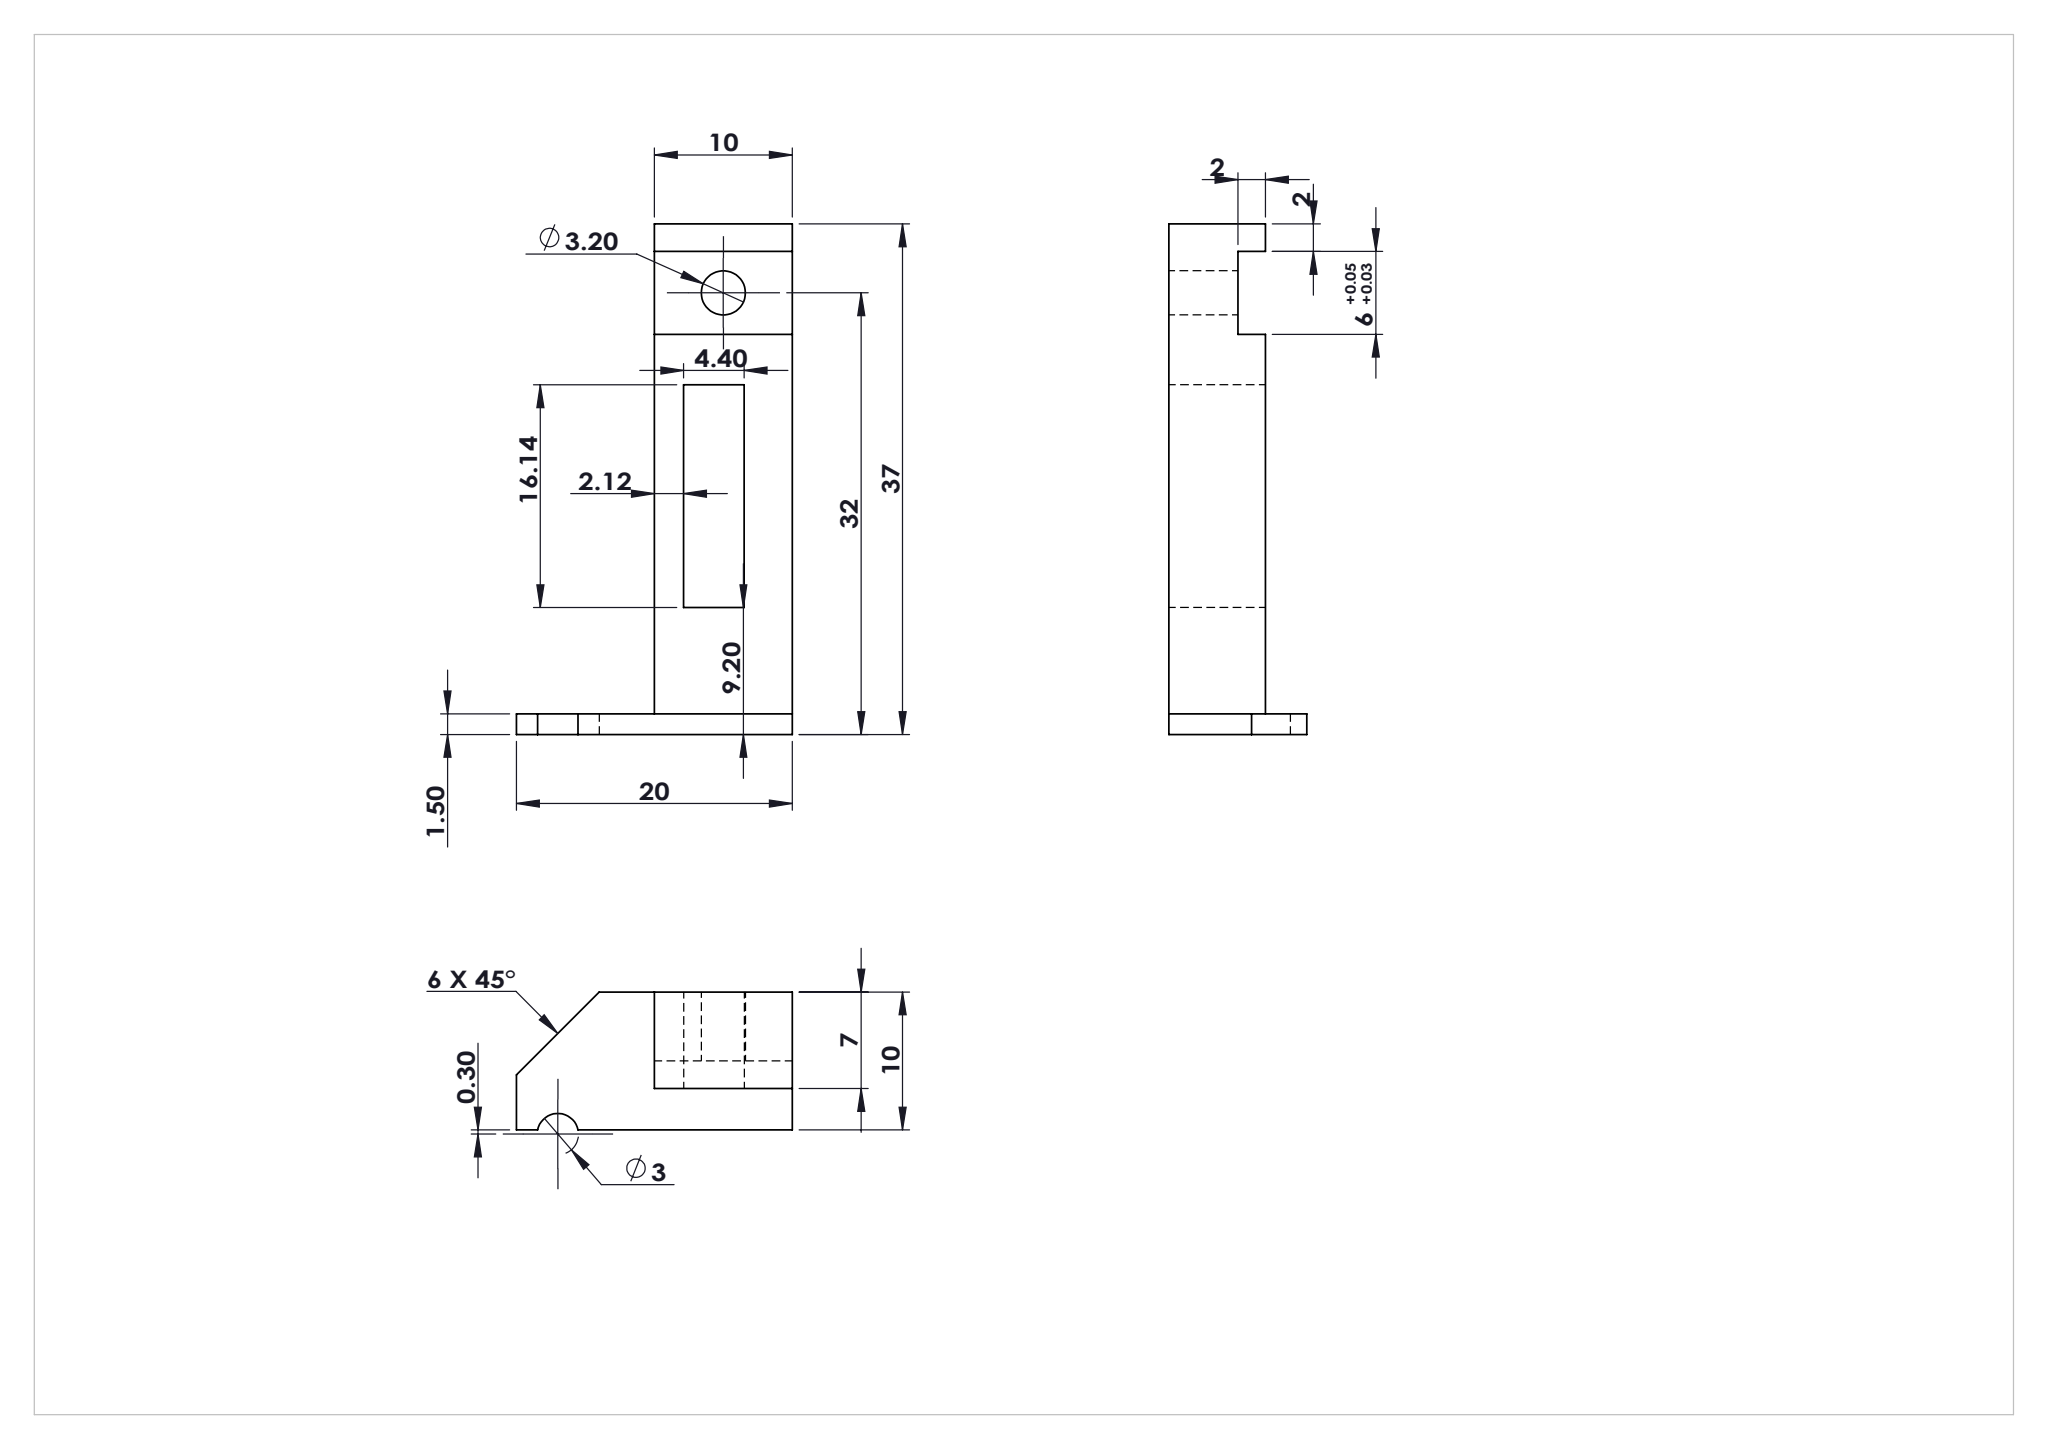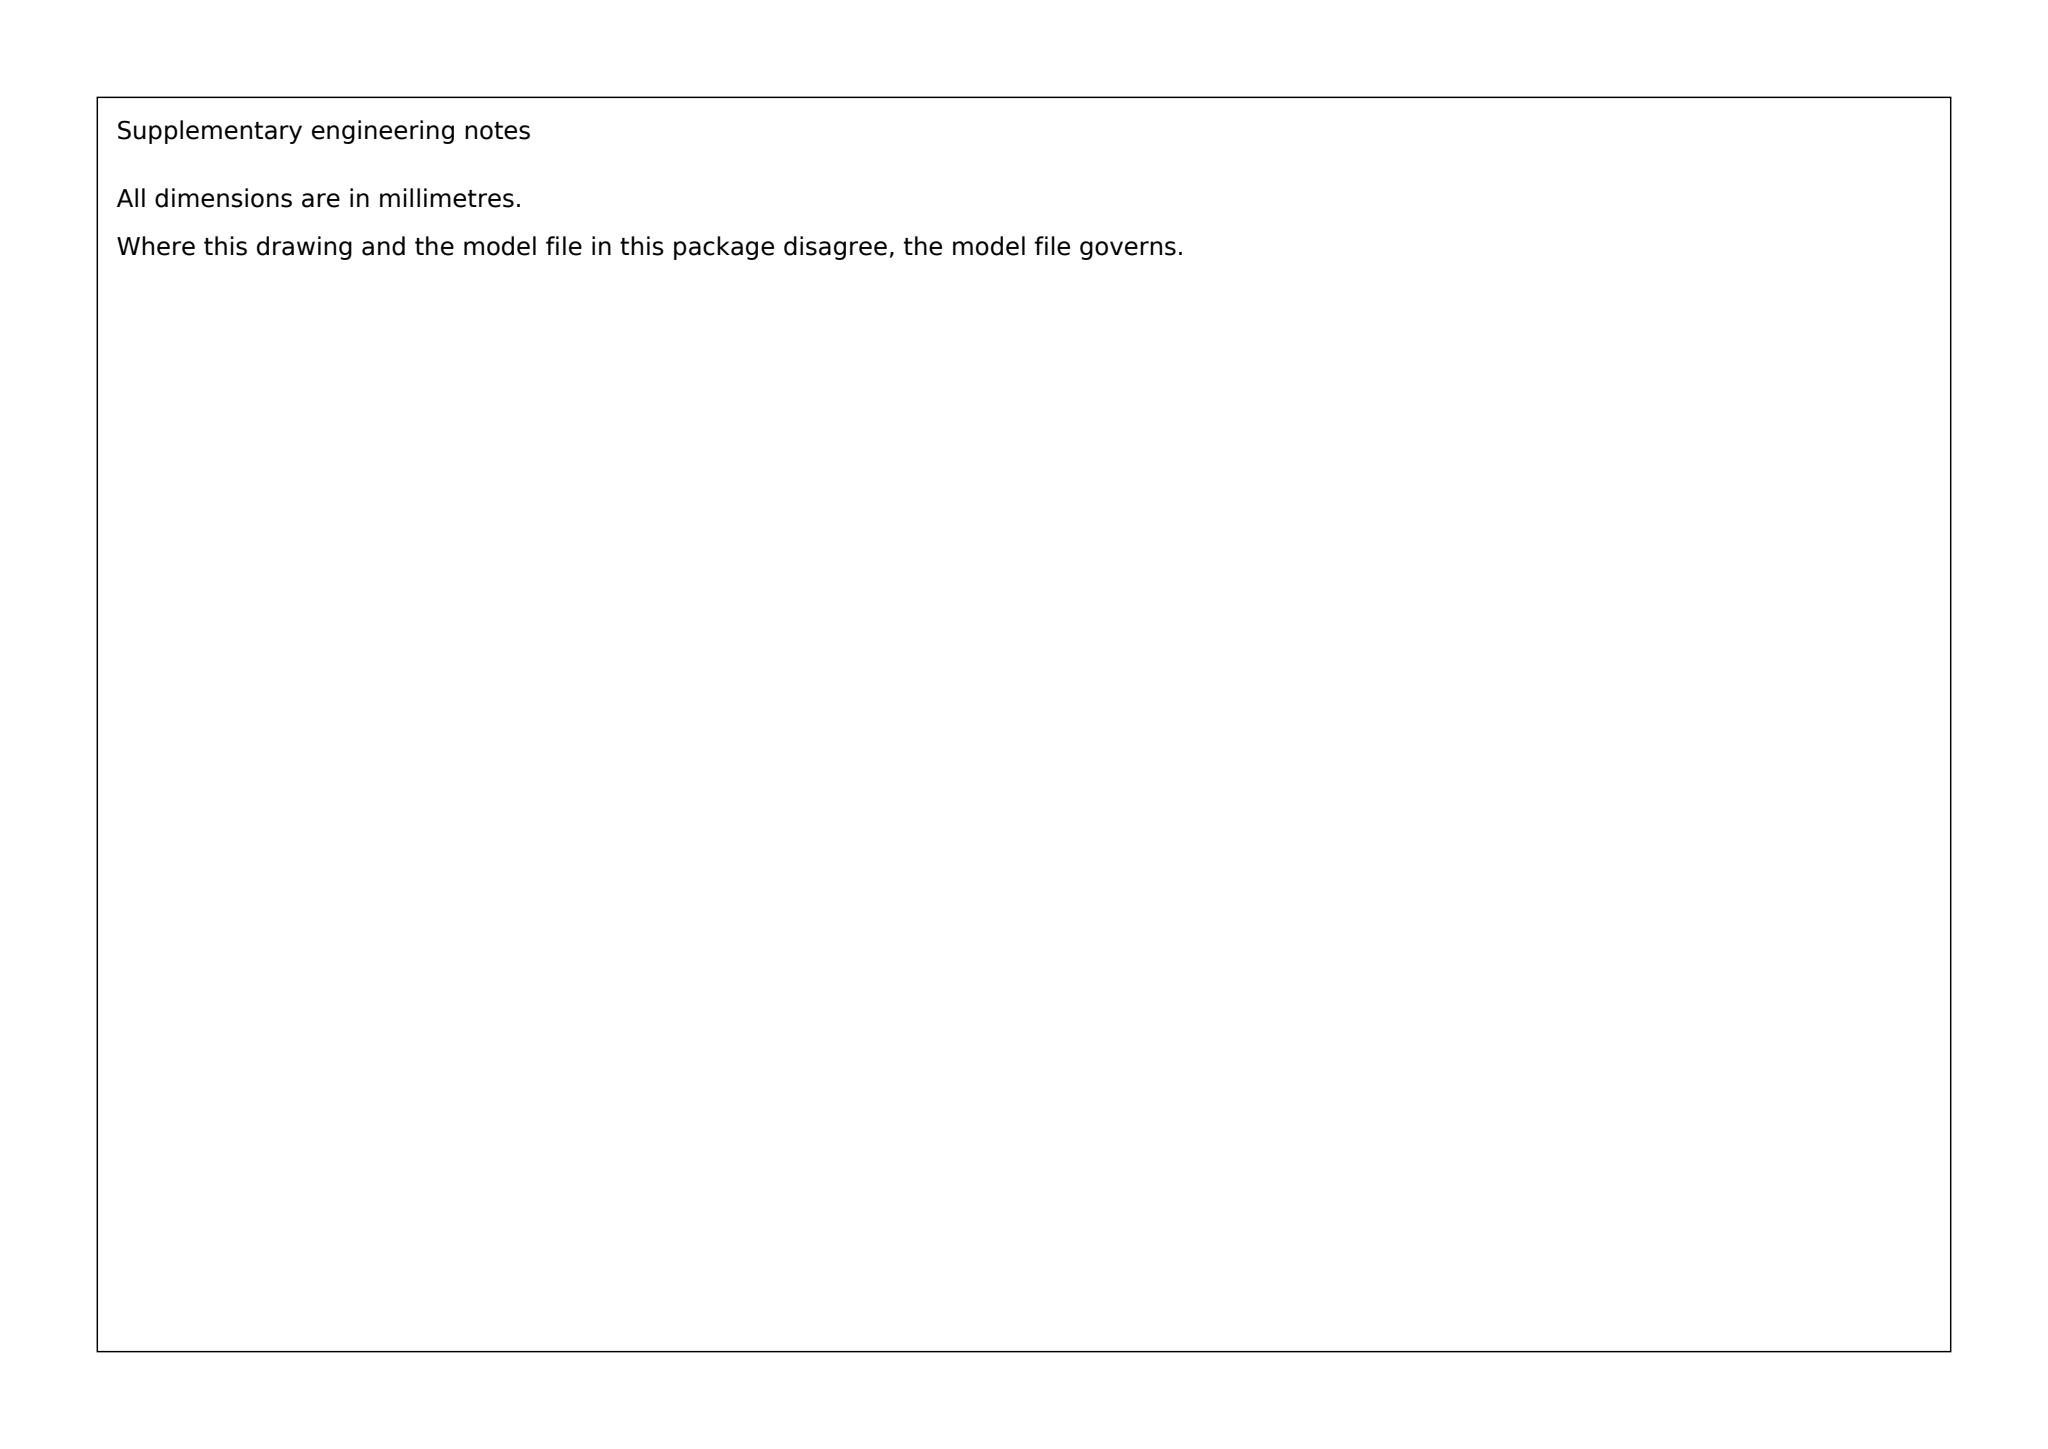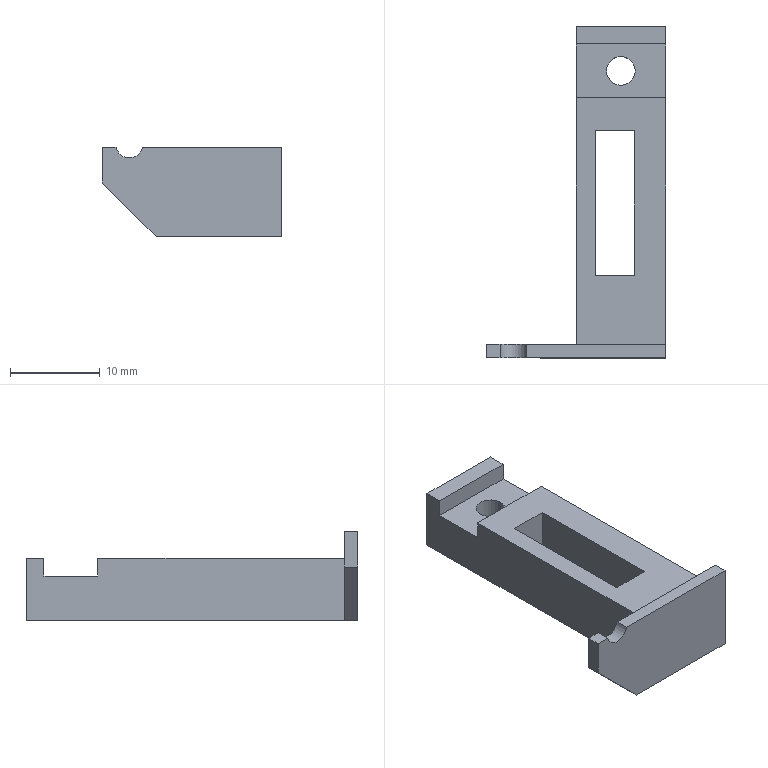Part | SolidWorks | mm | 1 solid | 22 faces | box 20 x 37 x 10 mm | volume 2097 mm3 | plane 19 | cylinder 3 | commonest cylinder face diameters 3.2 x2 3 x1
Drawing notes:
Ø3 HOLE IN BASE: AXIS 3 FROM LEFT END OF 20 BASE | from the solid: cylinder dia 3.0, axis y, pos x=3.0, z=10.3, len 1.5; bbox x=20
Ø3.20 HOLE ON CL OF 10 WIDE WALL: 5 FROM RH EDGE | from the solid: cyl Ø3.2 axis z at x=15.0; wall faces x=10.0 and x=20.0 -> 5 each side
RECTANGULAR POCKET 4.40 WIDE X 16.14 HIGH THRU VERTICAL WALL (WALL 7 THK); POCKET SIDES 12.12 AND 16.52 FROM LH END OF 20 BASE, BOTTOM 9.20 ABOVE BASE UNDERSIDE | from the solid: axis_planes x=12.12 & x=16.52, y=9.2 & y=25.34; no z plane between z=0 (back face) and z=7 (wall front face) inside pocket, i.e. pocket is open both sides = THRU
Ø3 HOLE THRU 1.50 THK BASE, AXIS 3 FROM LH END OF 20 BASE AND 10.30 FROM WALL BACK FACE (DATUM z=0) | from the solid: cylinders[3.0,"y",[3.0,null,10.3],1.5]
build123d program:
from build123d import *

# Parameters (mm, degrees)
SKETCH1_W            = 10
SKETCH1_H            = 37
BOSS_EXTRUDE1_DEPTH  = 10
SKETCH3_W            = 3
SKETCH3_H            = 35.5
CUT_EXTRUDE2_DEPTH   = 24.286
SKETCH7_W            = 10
SKETCH7_H            = 6
CUT_EXTRUDE6_DEPTH   = 2
SKETCH8_W            = 10
SKETCH8_H            = 1.5
BOSS_EXTRUDE2_DEPTH  = 10
SKETCH9_R            = 1.5
CUT_EXTRUDE7_DEPTH   = 40.815
CHAMFER1_SIZE        = 6
SKETCH1_2_R          = 1.6
CUT_EXTRUDE1_DEPTH   = 25.336
SKETCH2_W            = 4.395
SKETCH2_H            = 16.14
CUT_EXTRUDE2_2_DEPTH = 10


with BuildPart() as part:
    # Sketch1 → Boss-Extrude1 (new body)
    with BuildSketch(Plane.XY):
        Rectangle(SKETCH1_W, SKETCH1_H)
    extrude(amount=-BOSS_EXTRUDE1_DEPTH)

    # Sketch3 → Cut-Extrude2 (cut, through all)
    with BuildSketch(Plane(origin=(5, 0, 0), x_dir=(0, 0, -1), z_dir=(1, 0, 0))):
        with Locations((1.5, 0.75)):
            Rectangle(SKETCH3_W, SKETCH3_H)
    extrude(amount=-CUT_EXTRUDE2_DEPTH, mode=Mode.SUBTRACT)

    # Sketch7 → Cut-Extrude6 (cut)
    with BuildSketch(Plane.XY.offset(-3)):
        with Locations((0, 13.5)):
            Rectangle(SKETCH7_W, SKETCH7_H)
    extrude(amount=-CUT_EXTRUDE6_DEPTH, mode=Mode.SUBTRACT)

    # Sketch8 → Boss-Extrude2 (add)
    with BuildSketch(Plane.ZY.offset(5)):
        with Locations((-5, -17.75)):
            Rectangle(SKETCH8_W, SKETCH8_H)
    extrude(amount=BOSS_EXTRUDE2_DEPTH)

    # Sketch9 → Cut-Extrude7 (cut, through all)
    with BuildSketch(Plane(origin=(0, -17, 0), x_dir=(1, 0, 0), z_dir=(0, 1, 0))):
        with Locations((-12, -0.3)):
            Circle(SKETCH9_R)
    extrude(amount=-CUT_EXTRUDE7_DEPTH, mode=Mode.SUBTRACT)

    # Chamfer1
    chamfer1_edges = [part.edges().sort_by_distance(p)[0] for p in [
        (-15, -17.75, -10),
    ]]
    chamfer(chamfer1_edges, length=CHAMFER1_SIZE)

    # Sketch1_2 → Cut-Extrude1 (cut, through all)
    with BuildSketch(Plane.XY.offset(-5)):
        with Locations((0, 13.5)):
            Circle(SKETCH1_2_R)
    extrude(amount=-CUT_EXTRUDE1_DEPTH, mode=Mode.SUBTRACT)

    # Sketch2 → Cut-Extrude2_2 (cut)
    with BuildSketch(Plane.XY.offset(-3)):
        with Locations((-0.6807, -1.231)):
            Rectangle(SKETCH2_W, SKETCH2_H)
    extrude(amount=-CUT_EXTRUDE2_2_DEPTH, mode=Mode.SUBTRACT)


solid = part.part
STEP:
#1=CARTESIAN_POINT('',(-1.6,13.5,-10.));
#2=VERTEX_POINT('',#1);
#3=CARTESIAN_POINT('',(1.6,13.5,-10.));
#4=VERTEX_POINT('',#3);
#5=CARTESIAN_POINT('',(0.,13.5,-10.));
#6=DIRECTION('',(0.,0.,1.));
#7=DIRECTION('',(1.,0.,0.));
#8=AXIS2_PLACEMENT_3D('',#5,#6,#7);
#9=CIRCLE('',#8,1.6);
#10=EDGE_CURVE('',#2,#4,#9,.T.);
#11=ORIENTED_EDGE('',*,*,#10,.F.);
#12=CARTESIAN_POINT('',(-1.6,13.5,-5.));
#13=VERTEX_POINT('',#12);
#14=CARTESIAN_POINT('',(-1.6,13.5,-10.));
#15=DIRECTION('',(0.,0.,1.));
#16=VECTOR('',#15,1000.);
#17=LINE('',#14,#16);
#18=EDGE_CURVE('',#2,#13,#17,.T.);
#19=ORIENTED_EDGE('',*,*,#18,.T.);
#20=CARTESIAN_POINT('',(1.6,13.5,-5.));
#21=VERTEX_POINT('',#20);
#22=CARTESIAN_POINT('',(0.,13.5,-5.));
#23=DIRECTION('',(0.,0.,1.));
#24=DIRECTION('',(1.,0.,0.));
#25=AXIS2_PLACEMENT_3D('',#22,#23,#24);
#26=CIRCLE('',#25,1.6);
#27=EDGE_CURVE('',#13,#21,#26,.T.);
#28=ORIENTED_EDGE('',*,*,#27,.T.);
#29=CARTESIAN_POINT('',(1.6,13.5,-10.));
#30=DIRECTION('',(0.,0.,1.));
#31=VECTOR('',#30,1000.);
#32=LINE('',#29,#31);
#33=EDGE_CURVE('',#4,#21,#32,.T.);
#34=ORIENTED_EDGE('',*,*,#33,.F.);
#35=EDGE_LOOP('',(#11,#19,#28,#34));
#36=FACE_OUTER_BOUND('',#35,.T.);
#37=CARTESIAN_POINT('',(0.,13.5,-10.));
#38=DIRECTION('',(0.,0.,1.));
#39=DIRECTION('',(1.,0.,0.));
#40=AXIS2_PLACEMENT_3D('',#37,#38,#39);
#41=CYLINDRICAL_SURFACE('',#40,1.6);
#42=ADVANCED_FACE('',(#36),#41,.F.);
#43=CARTESIAN_POINT('',(-10.53,-18.5,0.));
#44=VERTEX_POINT('',#43);
#45=CARTESIAN_POINT('',(-10.53,-17.,-0.));
#46=VERTEX_POINT('',#45);
#47=CARTESIAN_POINT('',(-10.53,-18.5,0.));
#48=DIRECTION('',(0.,1.,-0.));
#49=VECTOR('',#48,1000.);
#50=LINE('',#47,#49);
#51=EDGE_CURVE('',#44,#46,#50,.T.);
#52=ORIENTED_EDGE('',*,*,#51,.F.);
#53=CARTESIAN_POINT('',(5.,-18.5,0.));
#54=VERTEX_POINT('',#53);
#55=CARTESIAN_POINT('',(5.,-18.5,0.));
#56=DIRECTION('',(1.,0.,0.));
#57=VECTOR('',#56,1000.);
#58=LINE('',#55,#57);
#59=EDGE_CURVE('',#44,#54,#58,.T.);
#60=ORIENTED_EDGE('',*,*,#59,.T.);
#61=CARTESIAN_POINT('',(5.,-17.,-0.));
#62=VERTEX_POINT('',#61);
#63=CARTESIAN_POINT('',(5.,-18.5,0.));
#64=DIRECTION('',(0.,1.,0.));
#65=VECTOR('',#64,1000.);
#66=LINE('',#63,#65);
#67=EDGE_CURVE('',#54,#62,#66,.T.);
#68=ORIENTED_EDGE('',*,*,#67,.T.);
#69=CARTESIAN_POINT('',(-5.,-17.,-0.));
#70=DIRECTION('',(1.,0.,0.));
#71=VECTOR('',#70,1000.);
#72=LINE('',#69,#71);
#73=EDGE_CURVE('',#46,#62,#72,.T.);
#74=ORIENTED_EDGE('',*,*,#73,.F.);
#75=EDGE_LOOP('',(#52,#60,#68,#74));
#76=FACE_OUTER_BOUND('',#75,.T.);
#77=CARTESIAN_POINT('',(0.,0.,0.));
#78=DIRECTION('',(0.,0.,1.));
#79=DIRECTION('',(1.,0.,0.));
#80=AXIS2_PLACEMENT_3D('',#77,#78,#79);
#81=PLANE('',#80);
#82=ADVANCED_FACE('',(#76),#81,.T.);
#83=CARTESIAN_POINT('',(-5.,16.5,-3.));
#84=VERTEX_POINT('',#83);
#85=CARTESIAN_POINT('',(-5.,18.5,-3.));
#86=VERTEX_POINT('',#85);
#87=CARTESIAN_POINT('',(-5.,18.5,-3.));
#88=DIRECTION('',(0.,1.,0.));
#89=VECTOR('',#88,1000.);
#90=LINE('',#87,#89);
#91=EDGE_CURVE('',#84,#86,#90,.T.);
#92=ORIENTED_EDGE('',*,*,#91,.F.);
#93=CARTESIAN_POINT('',(5.,16.5,-3.));
#94=VERTEX_POINT('',#93);
#95=CARTESIAN_POINT('',(-5.,16.5,-3.));
#96=DIRECTION('',(-1.,0.,0.));
#97=VECTOR('',#96,1000.);
#98=LINE('',#95,#97);
#99=EDGE_CURVE('',#94,#84,#98,.T.);
#100=ORIENTED_EDGE('',*,*,#99,.F.);
#101=CARTESIAN_POINT('',(5.,18.5,-3.));
#102=VERTEX_POINT('',#101);
#103=CARTESIAN_POINT('',(5.,18.5,-3.));
#104=DIRECTION('',(0.,1.,0.));
#105=VECTOR('',#104,1000.);
#106=LINE('',#103,#105);
#107=EDGE_CURVE('',#94,#102,#106,.T.);
#108=ORIENTED_EDGE('',*,*,#107,.T.);
#109=CARTESIAN_POINT('',(-5.,18.5,-3.));
#110=DIRECTION('',(1.,0.,0.));
#111=VECTOR('',#110,1000.);
#112=LINE('',#109,#111);
#113=EDGE_CURVE('',#86,#102,#112,.T.);
#114=ORIENTED_EDGE('',*,*,#113,.F.);
#115=EDGE_LOOP('',(#92,#100,#108,#114));
#116=FACE_OUTER_BOUND('',#115,.T.);
#117=CARTESIAN_POINT('',(-5.,18.5,-3.));
#118=DIRECTION('',(0.,0.,-1.));
#119=DIRECTION('',(0.,1.,0.));
#120=AXIS2_PLACEMENT_3D('',#117,#118,#119);
#121=PLANE('',#120);
#122=ADVANCED_FACE('',(#116),#121,.F.);
#123=CARTESIAN_POINT('',(-5.,-17.,-3.));
#124=VERTEX_POINT('',#123);
#125=CARTESIAN_POINT('',(-5.,-17.,-10.));
#126=VERTEX_POINT('',#125);
#127=CARTESIAN_POINT('',(-5.,-17.,0.));
#128=DIRECTION('',(0.,-0.,-1.));
#129=VECTOR('',#128,1000.);
#130=LINE('',#127,#129);
#131=EDGE_CURVE('',#124,#126,#130,.T.);
#132=ORIENTED_EDGE('',*,*,#131,.F.);
#133=CARTESIAN_POINT('',(-5.,10.5,-3.));
#134=VERTEX_POINT('',#133);
#135=CARTESIAN_POINT('',(-5.,18.5,-3.));
#136=DIRECTION('',(0.,1.,0.));
#137=VECTOR('',#136,1000.);
#138=LINE('',#135,#137);
#139=EDGE_CURVE('',#124,#134,#138,.T.);
#140=ORIENTED_EDGE('',*,*,#139,.T.);
#141=CARTESIAN_POINT('',(-5.,10.5,-5.));
#142=VERTEX_POINT('',#141);
#143=CARTESIAN_POINT('',(-5.,10.5,-5.));
#144=DIRECTION('',(0.,0.,1.));
#145=VECTOR('',#144,1000.);
#146=LINE('',#143,#145);
#147=EDGE_CURVE('',#142,#134,#146,.T.);
#148=ORIENTED_EDGE('',*,*,#147,.F.);
#149=CARTESIAN_POINT('',(-5.,16.5,-5.));
#150=VERTEX_POINT('',#149);
#151=CARTESIAN_POINT('',(-5.,16.5,-5.));
#152=DIRECTION('',(0.,-1.,0.));
#153=VECTOR('',#152,1000.);
#154=LINE('',#151,#153);
#155=EDGE_CURVE('',#150,#142,#154,.T.);
#156=ORIENTED_EDGE('',*,*,#155,.F.);
#157=CARTESIAN_POINT('',(-5.,16.5,-5.));
#158=DIRECTION('',(0.,0.,1.));
#159=VECTOR('',#158,1000.);
#160=LINE('',#157,#159);
#161=EDGE_CURVE('',#150,#84,#160,.T.);
#162=ORIENTED_EDGE('',*,*,#161,.T.);
#163=ORIENTED_EDGE('',*,*,#91,.T.);
#164=CARTESIAN_POINT('',(-5.,18.5,-10.));
#165=VERTEX_POINT('',#164);
#166=CARTESIAN_POINT('',(-5.,18.5,-10.));
#167=DIRECTION('',(0.,0.,1.));
#168=VECTOR('',#167,1000.);
#169=LINE('',#166,#168);
#170=EDGE_CURVE('',#165,#86,#169,.T.);
#171=ORIENTED_EDGE('',*,*,#170,.F.);
#172=CARTESIAN_POINT('',(-5.,-18.5,-10.));
#173=DIRECTION('',(0.,-1.,0.));
#174=VECTOR('',#173,1000.);
#175=LINE('',#172,#174);
#176=EDGE_CURVE('',#165,#126,#175,.T.);
#177=ORIENTED_EDGE('',*,*,#176,.T.);
#178=EDGE_LOOP('',(#132,#140,#148,#156,#162,#163,#171,#177));
#179=FACE_OUTER_BOUND('',#178,.T.);
#180=CARTESIAN_POINT('',(-5.,-18.5,-10.));
#181=DIRECTION('',(-1.,0.,0.));
#182=DIRECTION('',(0.,0.,1.));
#183=AXIS2_PLACEMENT_3D('',#180,#181,#182);
#184=PLANE('',#183);
#185=ADVANCED_FACE('',(#179),#184,.T.);
#186=ORIENTED_EDGE('',*,*,#113,.T.);
#187=CARTESIAN_POINT('',(5.,18.5,-10.));
#188=VERTEX_POINT('',#187);
#189=CARTESIAN_POINT('',(5.,18.5,-10.));
#190=DIRECTION('',(0.,0.,1.));
#191=VECTOR('',#190,1000.);
#192=LINE('',#189,#191);
#193=EDGE_CURVE('',#188,#102,#192,.T.);
#194=ORIENTED_EDGE('',*,*,#193,.F.);
#195=CARTESIAN_POINT('',(5.,18.5,-10.));
#196=DIRECTION('',(-1.,0.,0.));
#197=VECTOR('',#196,1000.);
#198=LINE('',#195,#197);
#199=EDGE_CURVE('',#188,#165,#198,.T.);
#200=ORIENTED_EDGE('',*,*,#199,.T.);
#201=ORIENTED_EDGE('',*,*,#170,.T.);
#202=EDGE_LOOP('',(#186,#194,#200,#201));
#203=FACE_OUTER_BOUND('',#202,.T.);
#204=CARTESIAN_POINT('',(5.,18.5,-10.));
#205=DIRECTION('',(0.,1.,0.));
#206=DIRECTION('',(0.,0.,1.));
#207=AXIS2_PLACEMENT_3D('',#204,#205,#206);
#208=PLANE('',#207);
#209=ADVANCED_FACE('',(#203),#208,.T.);
#210=CARTESIAN_POINT('',(5.,16.5,-5.));
#211=VERTEX_POINT('',#210);
#212=CARTESIAN_POINT('',(5.,16.5,-5.));
#213=DIRECTION('',(0.,0.,1.));
#214=VECTOR('',#213,1000.);
#215=LINE('',#212,#214);
#216=EDGE_CURVE('',#211,#94,#215,.T.);
#217=ORIENTED_EDGE('',*,*,#216,.F.);
#218=CARTESIAN_POINT('',(5.,10.5,-5.));
#219=VERTEX_POINT('',#218);
#220=CARTESIAN_POINT('',(5.,16.5,-5.));
#221=DIRECTION('',(-0.,1.,0.));
#222=VECTOR('',#221,1000.);
#223=LINE('',#220,#222);
#224=EDGE_CURVE('',#219,#211,#223,.T.);
#225=ORIENTED_EDGE('',*,*,#224,.F.);
#226=CARTESIAN_POINT('',(5.,10.5,-3.));
#227=VERTEX_POINT('',#226);
#228=CARTESIAN_POINT('',(5.,10.5,-5.));
#229=DIRECTION('',(0.,0.,1.));
#230=VECTOR('',#229,1000.);
#231=LINE('',#228,#230);
#232=EDGE_CURVE('',#219,#227,#231,.T.);
#233=ORIENTED_EDGE('',*,*,#232,.T.);
#234=CARTESIAN_POINT('',(5.,-17.,-3.));
#235=VERTEX_POINT('',#234);
#236=CARTESIAN_POINT('',(5.,18.5,-3.));
#237=DIRECTION('',(0.,1.,0.));
#238=VECTOR('',#237,1000.);
#239=LINE('',#236,#238);
#240=EDGE_CURVE('',#235,#227,#239,.T.);
#241=ORIENTED_EDGE('',*,*,#240,.F.);
#242=CARTESIAN_POINT('',(5.,-17.,-0.));
#243=DIRECTION('',(0.,0.,-1.));
#244=VECTOR('',#243,1000.);
#245=LINE('',#242,#244);
#246=EDGE_CURVE('',#62,#235,#245,.T.);
#247=ORIENTED_EDGE('',*,*,#246,.F.);
#248=ORIENTED_EDGE('',*,*,#67,.F.);
#249=CARTESIAN_POINT('',(5.,-18.5,-10.));
#250=VERTEX_POINT('',#249);
#251=CARTESIAN_POINT('',(5.,-18.5,-10.));
#252=DIRECTION('',(0.,0.,1.));
#253=VECTOR('',#252,1000.);
#254=LINE('',#251,#253);
#255=EDGE_CURVE('',#250,#54,#254,.T.);
#256=ORIENTED_EDGE('',*,*,#255,.F.);
#257=CARTESIAN_POINT('',(5.,-18.5,-10.));
#258=DIRECTION('',(0.,1.,0.));
#259=VECTOR('',#258,1000.);
#260=LINE('',#257,#259);
#261=EDGE_CURVE('',#250,#188,#260,.T.);
#262=ORIENTED_EDGE('',*,*,#261,.T.);
#263=ORIENTED_EDGE('',*,*,#193,.T.);
#264=ORIENTED_EDGE('',*,*,#107,.F.);
#265=EDGE_LOOP('',(#217,#225,#233,#241,#247,#248,#256,#262,#263,#264));
#266=FACE_OUTER_BOUND('',#265,.T.);
#267=CARTESIAN_POINT('',(5.,-18.5,-10.));
#268=DIRECTION('',(1.,0.,0.));
#269=DIRECTION('',(0.,0.,-1.));
#270=AXIS2_PLACEMENT_3D('',#267,#268,#269);
#271=PLANE('',#270);
#272=ADVANCED_FACE('',(#266),#271,.T.);
#273=CARTESIAN_POINT('',(-15.,-18.5,-4.));
#274=VERTEX_POINT('',#273);
#275=CARTESIAN_POINT('',(-15.,-18.5,0.));
#276=VERTEX_POINT('',#275);
#277=CARTESIAN_POINT('',(-15.,-18.5,0.));
#278=DIRECTION('',(0.,-0.,1.));
#279=VECTOR('',#278,1000.);
#280=LINE('',#277,#279);
#281=EDGE_CURVE('',#274,#276,#280,.T.);
#282=ORIENTED_EDGE('',*,*,#281,.F.);
#283=CARTESIAN_POINT('',(-9.,-18.5,-10.));
#284=VERTEX_POINT('',#283);
#285=CARTESIAN_POINT('',(-2.,-18.5,-17.));
#286=DIRECTION('',(0.7071,0.,-0.7071));
#287=VECTOR('',#286,1000.);
#288=LINE('',#285,#287);
#289=EDGE_CURVE('',#274,#284,#288,.T.);
#290=ORIENTED_EDGE('',*,*,#289,.T.);
#291=CARTESIAN_POINT('',(5.,-18.5,-10.));
#292=DIRECTION('',(1.,0.,0.));
#293=VECTOR('',#292,1000.);
#294=LINE('',#291,#293);
#295=EDGE_CURVE('',#284,#250,#294,.T.);
#296=ORIENTED_EDGE('',*,*,#295,.T.);
#297=ORIENTED_EDGE('',*,*,#255,.T.);
#298=ORIENTED_EDGE('',*,*,#59,.F.);
#299=CARTESIAN_POINT('',(-13.47,-18.5,0.));
#300=VERTEX_POINT('',#299);
#301=CARTESIAN_POINT('',(-12.,-18.5,0.3));
#302=DIRECTION('',(0.,1.,-0.));
#303=DIRECTION('',(0.,0.,1.));
#304=AXIS2_PLACEMENT_3D('',#301,#302,#303);
#305=CIRCLE('',#304,1.5);
#306=EDGE_CURVE('',#44,#300,#305,.T.);
#307=ORIENTED_EDGE('',*,*,#306,.T.);
#308=CARTESIAN_POINT('',(5.,-18.5,0.));
#309=DIRECTION('',(1.,0.,0.));
#310=VECTOR('',#309,1000.);
#311=LINE('',#308,#310);
#312=EDGE_CURVE('',#276,#300,#311,.T.);
#313=ORIENTED_EDGE('',*,*,#312,.F.);
#314=EDGE_LOOP('',(#282,#290,#296,#297,#298,#307,#313));
#315=FACE_OUTER_BOUND('',#314,.T.);
#316=CARTESIAN_POINT('',(5.,-18.5,-10.));
#317=DIRECTION('',(0.,-1.,0.));
#318=DIRECTION('',(0.,0.,-1.));
#319=AXIS2_PLACEMENT_3D('',#316,#317,#318);
#320=PLANE('',#319);
#321=ADVANCED_FACE('',(#315),#320,.T.);
#322=CARTESIAN_POINT('',(1.517,6.839,-10.));
#323=VERTEX_POINT('',#322);
#324=CARTESIAN_POINT('',(-2.878,6.839,-10.));
#325=VERTEX_POINT('',#324);
#326=CARTESIAN_POINT('',(0.,6.839,-10.));
#327=DIRECTION('',(-1.,0.,0.));
#328=VECTOR('',#327,1000.);
#329=LINE('',#326,#328);
#330=EDGE_CURVE('',#323,#325,#329,.T.);
#331=ORIENTED_EDGE('',*,*,#330,.T.);
#332=CARTESIAN_POINT('',(-2.878,-9.302,-10.));
#333=VERTEX_POINT('',#332);
#334=CARTESIAN_POINT('',(-2.878,0.,-10.));
#335=DIRECTION('',(0.,-1.,0.));
#336=VECTOR('',#335,1000.);
#337=LINE('',#334,#336);
#338=EDGE_CURVE('',#325,#333,#337,.T.);
#339=ORIENTED_EDGE('',*,*,#338,.T.);
#340=CARTESIAN_POINT('',(1.517,-9.302,-10.));
#341=VERTEX_POINT('',#340);
#342=CARTESIAN_POINT('',(0.,-9.302,-10.));
#343=DIRECTION('',(1.,0.,0.));
#344=VECTOR('',#343,1000.);
#345=LINE('',#342,#344);
#346=EDGE_CURVE('',#333,#341,#345,.T.);
#347=ORIENTED_EDGE('',*,*,#346,.T.);
#348=CARTESIAN_POINT('',(1.517,0.,-10.));
#349=DIRECTION('',(0.,1.,0.));
#350=VECTOR('',#349,1000.);
#351=LINE('',#348,#350);
#352=EDGE_CURVE('',#341,#323,#351,.T.);
#353=ORIENTED_EDGE('',*,*,#352,.T.);
#354=EDGE_LOOP('',(#331,#339,#347,#353));
#355=FACE_BOUND('',#354,.T.);
#356=CARTESIAN_POINT('',(0.,13.5,-10.));
#357=DIRECTION('',(0.,0.,1.));
#358=DIRECTION('',(1.,0.,0.));
#359=AXIS2_PLACEMENT_3D('',#356,#357,#358);
#360=CIRCLE('',#359,1.6);
#361=EDGE_CURVE('',#4,#2,#360,.T.);
#362=ORIENTED_EDGE('',*,*,#361,.T.);
#363=ORIENTED_EDGE('',*,*,#10,.T.);
#364=EDGE_LOOP('',(#362,#363));
#365=FACE_BOUND('',#364,.T.);
#366=ORIENTED_EDGE('',*,*,#295,.F.);
#367=CARTESIAN_POINT('',(-9.,-17.,-10.));
#368=VERTEX_POINT('',#367);
#369=CARTESIAN_POINT('',(-9.,0.,-10.));
#370=DIRECTION('',(0.,1.,0.));
#371=VECTOR('',#370,1000.);
#372=LINE('',#369,#371);
#373=EDGE_CURVE('',#284,#368,#372,.T.);
#374=ORIENTED_EDGE('',*,*,#373,.T.);
#375=CARTESIAN_POINT('',(-15.,-17.,-10.));
#376=DIRECTION('',(1.,0.,0.));
#377=VECTOR('',#376,1000.);
#378=LINE('',#375,#377);
#379=EDGE_CURVE('',#368,#126,#378,.T.);
#380=ORIENTED_EDGE('',*,*,#379,.T.);
#381=ORIENTED_EDGE('',*,*,#176,.F.);
#382=ORIENTED_EDGE('',*,*,#199,.F.);
#383=ORIENTED_EDGE('',*,*,#261,.F.);
#384=EDGE_LOOP('',(#366,#374,#380,#381,#382,#383));
#385=FACE_OUTER_BOUND('',#384,.T.);
#386=CARTESIAN_POINT('',(0.,0.,-10.));
#387=DIRECTION('',(0.,0.,1.));
#388=DIRECTION('',(1.,0.,0.));
#389=AXIS2_PLACEMENT_3D('',#386,#387,#388);
#390=PLANE('',#389);
#391=ADVANCED_FACE('',(#355,#365,#385),#390,.F.);
#392=CARTESIAN_POINT('',(-13.47,-17.,-0.));
#393=VERTEX_POINT('',#392);
#394=CARTESIAN_POINT('',(-13.47,-18.5,0.));
#395=DIRECTION('',(0.,-1.,0.));
#396=VECTOR('',#395,1000.);
#397=LINE('',#394,#396);
#398=EDGE_CURVE('',#393,#300,#397,.T.);
#399=ORIENTED_EDGE('',*,*,#398,.F.);
#400=CARTESIAN_POINT('',(-15.,-17.,0.));
#401=VERTEX_POINT('',#400);
#402=CARTESIAN_POINT('',(-5.,-17.,-0.));
#403=DIRECTION('',(1.,0.,0.));
#404=VECTOR('',#403,1000.);
#405=LINE('',#402,#404);
#406=EDGE_CURVE('',#401,#393,#405,.T.);
#407=ORIENTED_EDGE('',*,*,#406,.F.);
#408=CARTESIAN_POINT('',(-15.,-17.,0.));
#409=DIRECTION('',(0.,1.,-0.));
#410=VECTOR('',#409,1000.);
#411=LINE('',#408,#410);
#412=EDGE_CURVE('',#276,#401,#411,.T.);
#413=ORIENTED_EDGE('',*,*,#412,.F.);
#414=ORIENTED_EDGE('',*,*,#312,.T.);
#415=EDGE_LOOP('',(#399,#407,#413,#414));
#416=FACE_OUTER_BOUND('',#415,.T.);
#417=CARTESIAN_POINT('',(0.,0.,0.));
#418=DIRECTION('',(0.,0.,1.));
#419=DIRECTION('',(1.,0.,0.));
#420=AXIS2_PLACEMENT_3D('',#417,#418,#419);
#421=PLANE('',#420);
#422=ADVANCED_FACE('',(#416),#421,.T.);
#423=CARTESIAN_POINT('',(-2.878,-9.302,-3.));
#424=VERTEX_POINT('',#423);
#425=CARTESIAN_POINT('',(1.517,-9.302,-3.));
#426=VERTEX_POINT('',#425);
#427=CARTESIAN_POINT('',(-2.878,-9.302,-3.));
#428=DIRECTION('',(1.,0.,0.));
#429=VECTOR('',#428,1000.);
#430=LINE('',#427,#429);
#431=EDGE_CURVE('',#424,#426,#430,.T.);
#432=ORIENTED_EDGE('',*,*,#431,.F.);
#433=CARTESIAN_POINT('',(-2.878,6.839,-3.));
#434=VERTEX_POINT('',#433);
#435=CARTESIAN_POINT('',(-2.878,6.839,-3.));
#436=DIRECTION('',(0.,-1.,0.));
#437=VECTOR('',#436,1000.);
#438=LINE('',#435,#437);
#439=EDGE_CURVE('',#434,#424,#438,.T.);
#440=ORIENTED_EDGE('',*,*,#439,.F.);
#441=CARTESIAN_POINT('',(1.517,6.839,-3.));
#442=VERTEX_POINT('',#441);
#443=CARTESIAN_POINT('',(-2.878,6.839,-3.));
#444=DIRECTION('',(-1.,0.,0.));
#445=VECTOR('',#444,1000.);
#446=LINE('',#443,#445);
#447=EDGE_CURVE('',#442,#434,#446,.T.);
#448=ORIENTED_EDGE('',*,*,#447,.F.);
#449=CARTESIAN_POINT('',(1.517,6.839,-3.));
#450=DIRECTION('',(0.,1.,0.));
#451=VECTOR('',#450,1000.);
#452=LINE('',#449,#451);
#453=EDGE_CURVE('',#426,#442,#452,.T.);
#454=ORIENTED_EDGE('',*,*,#453,.F.);
#455=EDGE_LOOP('',(#432,#440,#448,#454));
#456=FACE_BOUND('',#455,.T.);
#457=ORIENTED_EDGE('',*,*,#240,.T.);
#458=CARTESIAN_POINT('',(-5.,10.5,-3.));
#459=DIRECTION('',(1.,-0.,0.));
#460=VECTOR('',#459,1000.);
#461=LINE('',#458,#460);
#462=EDGE_CURVE('',#134,#227,#461,.T.);
#463=ORIENTED_EDGE('',*,*,#462,.F.);
#464=ORIENTED_EDGE('',*,*,#139,.F.);
#465=CARTESIAN_POINT('',(-5.,-17.,-3.));
#466=DIRECTION('',(1.,0.,0.));
#467=VECTOR('',#466,1000.);
#468=LINE('',#465,#467);
#469=EDGE_CURVE('',#124,#235,#468,.T.);
#470=ORIENTED_EDGE('',*,*,#469,.T.);
#471=EDGE_LOOP('',(#457,#463,#464,#470));
#472=FACE_OUTER_BOUND('',#471,.T.);
#473=CARTESIAN_POINT('',(-5.,18.5,-3.));
#474=DIRECTION('',(0.,0.,-1.));
#475=DIRECTION('',(0.,1.,0.));
#476=AXIS2_PLACEMENT_3D('',#473,#474,#475);
#477=PLANE('',#476);
#478=ADVANCED_FACE('',(#456,#472),#477,.F.);
#479=ORIENTED_EDGE('',*,*,#379,.F.);
#480=CARTESIAN_POINT('',(-15.,-17.,-4.));
#481=VERTEX_POINT('',#480);
#482=CARTESIAN_POINT('',(-15.,-17.,-4.));
#483=DIRECTION('',(-0.7071,0.,0.7071));
#484=VECTOR('',#483,1000.);
#485=LINE('',#482,#484);
#486=EDGE_CURVE('',#368,#481,#485,.T.);
#487=ORIENTED_EDGE('',*,*,#486,.T.);
#488=CARTESIAN_POINT('',(-15.,-17.,0.));
#489=DIRECTION('',(0.,-0.,-1.));
#490=VECTOR('',#489,1000.);
#491=LINE('',#488,#490);
#492=EDGE_CURVE('',#401,#481,#491,.T.);
#493=ORIENTED_EDGE('',*,*,#492,.F.);
#494=ORIENTED_EDGE('',*,*,#406,.T.);
#495=CARTESIAN_POINT('',(-12.,-17.,0.3));
#496=DIRECTION('',(0.,1.,-0.));
#497=DIRECTION('',(0.,0.,1.));
#498=AXIS2_PLACEMENT_3D('',#495,#496,#497);
#499=CIRCLE('',#498,1.5);
#500=EDGE_CURVE('',#46,#393,#499,.T.);
#501=ORIENTED_EDGE('',*,*,#500,.F.);
#502=ORIENTED_EDGE('',*,*,#73,.T.);
#503=ORIENTED_EDGE('',*,*,#246,.T.);
#504=ORIENTED_EDGE('',*,*,#469,.F.);
#505=ORIENTED_EDGE('',*,*,#131,.T.);
#506=EDGE_LOOP('',(#479,#487,#493,#494,#501,#502,#503,#504,#505));
#507=FACE_OUTER_BOUND('',#506,.T.);
#508=CARTESIAN_POINT('',(-5.,-17.,-0.));
#509=DIRECTION('',(0.,-1.,0.));
#510=DIRECTION('',(0.,0.,-1.));
#511=AXIS2_PLACEMENT_3D('',#508,#509,#510);
#512=PLANE('',#511);
#513=ADVANCED_FACE('',(#507),#512,.F.);
#514=ORIENTED_EDGE('',*,*,#99,.T.);
#515=ORIENTED_EDGE('',*,*,#161,.F.);
#516=CARTESIAN_POINT('',(-5.,16.5,-5.));
#517=DIRECTION('',(-1.,0.,0.));
#518=VECTOR('',#517,1000.);
#519=LINE('',#516,#518);
#520=EDGE_CURVE('',#211,#150,#519,.T.);
#521=ORIENTED_EDGE('',*,*,#520,.F.);
#522=ORIENTED_EDGE('',*,*,#216,.T.);
#523=EDGE_LOOP('',(#514,#515,#521,#522));
#524=FACE_OUTER_BOUND('',#523,.T.);
#525=CARTESIAN_POINT('',(-5.,16.5,-5.));
#526=DIRECTION('',(0.,1.,0.));
#527=DIRECTION('',(0.,0.,1.));
#528=AXIS2_PLACEMENT_3D('',#525,#526,#527);
#529=PLANE('',#528);
#530=ADVANCED_FACE('',(#524),#529,.F.);
#531=ORIENTED_EDGE('',*,*,#462,.T.);
#532=ORIENTED_EDGE('',*,*,#232,.F.);
#533=CARTESIAN_POINT('',(-5.,10.5,-5.));
#534=DIRECTION('',(1.,-0.,0.));
#535=VECTOR('',#534,1000.);
#536=LINE('',#533,#535);
#537=EDGE_CURVE('',#142,#219,#536,.T.);
#538=ORIENTED_EDGE('',*,*,#537,.F.);
#539=ORIENTED_EDGE('',*,*,#147,.T.);
#540=EDGE_LOOP('',(#531,#532,#538,#539));
#541=FACE_OUTER_BOUND('',#540,.T.);
#542=CARTESIAN_POINT('',(-5.,10.5,-5.));
#543=DIRECTION('',(-0.,-1.,0.));
#544=DIRECTION('',(1.,-0.,0.));
#545=AXIS2_PLACEMENT_3D('',#542,#543,#544);
#546=PLANE('',#545);
#547=ADVANCED_FACE('',(#541),#546,.F.);
#548=CARTESIAN_POINT('',(0.,13.5,-5.));
#549=DIRECTION('',(0.,0.,1.));
#550=DIRECTION('',(1.,0.,0.));
#551=AXIS2_PLACEMENT_3D('',#548,#549,#550);
#552=CIRCLE('',#551,1.6);
#553=EDGE_CURVE('',#21,#13,#552,.T.);
#554=ORIENTED_EDGE('',*,*,#553,.F.);
#555=ORIENTED_EDGE('',*,*,#27,.F.);
#556=EDGE_LOOP('',(#554,#555));
#557=FACE_BOUND('',#556,.T.);
#558=ORIENTED_EDGE('',*,*,#155,.T.);
#559=ORIENTED_EDGE('',*,*,#537,.T.);
#560=ORIENTED_EDGE('',*,*,#224,.T.);
#561=ORIENTED_EDGE('',*,*,#520,.T.);
#562=EDGE_LOOP('',(#558,#559,#560,#561));
#563=FACE_OUTER_BOUND('',#562,.T.);
#564=CARTESIAN_POINT('',(0.,0.,-5.));
#565=DIRECTION('',(0.,0.,1.));
#566=DIRECTION('',(1.,0.,0.));
#567=AXIS2_PLACEMENT_3D('',#564,#565,#566);
#568=PLANE('',#567);
#569=ADVANCED_FACE('',(#557,#563),#568,.T.);
#570=ORIENTED_EDGE('',*,*,#492,.T.);
#571=CARTESIAN_POINT('',(-15.,0.,-4.));
#572=DIRECTION('',(0.,-1.,0.));
#573=VECTOR('',#572,1000.);
#574=LINE('',#571,#573);
#575=EDGE_CURVE('',#481,#274,#574,.T.);
#576=ORIENTED_EDGE('',*,*,#575,.T.);
#577=ORIENTED_EDGE('',*,*,#281,.T.);
#578=ORIENTED_EDGE('',*,*,#412,.T.);
#579=EDGE_LOOP('',(#570,#576,#577,#578));
#580=FACE_OUTER_BOUND('',#579,.T.);
#581=CARTESIAN_POINT('',(-15.,0.,0.));
#582=DIRECTION('',(1.,0.,0.));
#583=DIRECTION('',(0.,0.,-1.));
#584=AXIS2_PLACEMENT_3D('',#581,#582,#583);
#585=PLANE('',#584);
#586=ADVANCED_FACE('',(#580),#585,.F.);
#587=ORIENTED_EDGE('',*,*,#51,.T.);
#588=ORIENTED_EDGE('',*,*,#500,.T.);
#589=ORIENTED_EDGE('',*,*,#398,.T.);
#590=ORIENTED_EDGE('',*,*,#306,.F.);
#591=EDGE_LOOP('',(#587,#588,#589,#590));
#592=FACE_OUTER_BOUND('',#591,.T.);
#593=CARTESIAN_POINT('',(-12.,-18.5,0.3));
#594=DIRECTION('',(0.,1.,-0.));
#595=DIRECTION('',(0.,0.,1.));
#596=AXIS2_PLACEMENT_3D('',#593,#594,#595);
#597=CYLINDRICAL_SURFACE('',#596,1.5);
#598=ADVANCED_FACE('',(#592),#597,.F.);
#599=ORIENTED_EDGE('',*,*,#486,.F.);
#600=ORIENTED_EDGE('',*,*,#373,.F.);
#601=ORIENTED_EDGE('',*,*,#289,.F.);
#602=ORIENTED_EDGE('',*,*,#575,.F.);
#603=EDGE_LOOP('',(#599,#600,#601,#602));
#604=FACE_OUTER_BOUND('',#603,.T.);
#605=CARTESIAN_POINT('',(-15.,0.,-4.));
#606=DIRECTION('',(0.7071,0.,0.7071));
#607=DIRECTION('',(0.,-1.,0.));
#608=AXIS2_PLACEMENT_3D('',#605,#606,#607);
#609=PLANE('',#608);
#610=ADVANCED_FACE('',(#604),#609,.F.);
#611=ORIENTED_EDGE('',*,*,#18,.F.);
#612=ORIENTED_EDGE('',*,*,#361,.F.);
#613=ORIENTED_EDGE('',*,*,#33,.T.);
#614=ORIENTED_EDGE('',*,*,#553,.T.);
#615=EDGE_LOOP('',(#611,#612,#613,#614));
#616=FACE_OUTER_BOUND('',#615,.T.);
#617=CARTESIAN_POINT('',(0.,13.5,-10.));
#618=DIRECTION('',(0.,0.,1.));
#619=DIRECTION('',(1.,0.,0.));
#620=AXIS2_PLACEMENT_3D('',#617,#618,#619);
#621=CYLINDRICAL_SURFACE('',#620,1.6);
#622=ADVANCED_FACE('',(#616),#621,.F.);
#623=CARTESIAN_POINT('',(-2.878,6.839,-13.));
#624=DIRECTION('',(0.,0.,1.));
#625=VECTOR('',#624,1000.);
#626=LINE('',#623,#625);
#627=EDGE_CURVE('',#325,#434,#626,.T.);
#628=ORIENTED_EDGE('',*,*,#627,.T.);
#629=ORIENTED_EDGE('',*,*,#439,.T.);
#630=CARTESIAN_POINT('',(-2.878,-9.302,-13.));
#631=DIRECTION('',(0.,0.,1.));
#632=VECTOR('',#631,1000.);
#633=LINE('',#630,#632);
#634=EDGE_CURVE('',#333,#424,#633,.T.);
#635=ORIENTED_EDGE('',*,*,#634,.F.);
#636=ORIENTED_EDGE('',*,*,#338,.F.);
#637=EDGE_LOOP('',(#628,#629,#635,#636));
#638=FACE_OUTER_BOUND('',#637,.T.);
#639=CARTESIAN_POINT('',(-2.878,6.839,-13.));
#640=DIRECTION('',(-1.,0.,0.));
#641=DIRECTION('',(0.,0.,1.));
#642=AXIS2_PLACEMENT_3D('',#639,#640,#641);
#643=PLANE('',#642);
#644=ADVANCED_FACE('',(#638),#643,.F.);
#645=CARTESIAN_POINT('',(1.517,6.839,-13.));
#646=DIRECTION('',(0.,0.,1.));
#647=VECTOR('',#646,1000.);
#648=LINE('',#645,#647);
#649=EDGE_CURVE('',#323,#442,#648,.T.);
#650=ORIENTED_EDGE('',*,*,#649,.T.);
#651=ORIENTED_EDGE('',*,*,#447,.T.);
#652=ORIENTED_EDGE('',*,*,#627,.F.);
#653=ORIENTED_EDGE('',*,*,#330,.F.);
#654=EDGE_LOOP('',(#650,#651,#652,#653));
#655=FACE_OUTER_BOUND('',#654,.T.);
#656=CARTESIAN_POINT('',(-2.878,6.839,-13.));
#657=DIRECTION('',(0.,1.,0.));
#658=DIRECTION('',(0.,0.,1.));
#659=AXIS2_PLACEMENT_3D('',#656,#657,#658);
#660=PLANE('',#659);
#661=ADVANCED_FACE('',(#655),#660,.F.);
#662=CARTESIAN_POINT('',(1.517,-9.302,-13.));
#663=DIRECTION('',(0.,0.,1.));
#664=VECTOR('',#663,1000.);
#665=LINE('',#662,#664);
#666=EDGE_CURVE('',#341,#426,#665,.T.);
#667=ORIENTED_EDGE('',*,*,#666,.T.);
#668=ORIENTED_EDGE('',*,*,#453,.T.);
#669=ORIENTED_EDGE('',*,*,#649,.F.);
#670=ORIENTED_EDGE('',*,*,#352,.F.);
#671=EDGE_LOOP('',(#667,#668,#669,#670));
#672=FACE_OUTER_BOUND('',#671,.T.);
#673=CARTESIAN_POINT('',(1.517,6.839,-13.));
#674=DIRECTION('',(1.,0.,0.));
#675=DIRECTION('',(0.,0.,-1.));
#676=AXIS2_PLACEMENT_3D('',#673,#674,#675);
#677=PLANE('',#676);
#678=ADVANCED_FACE('',(#672),#677,.F.);
#679=ORIENTED_EDGE('',*,*,#634,.T.);
#680=ORIENTED_EDGE('',*,*,#431,.T.);
#681=ORIENTED_EDGE('',*,*,#666,.F.);
#682=ORIENTED_EDGE('',*,*,#346,.F.);
#683=EDGE_LOOP('',(#679,#680,#681,#682));
#684=FACE_OUTER_BOUND('',#683,.T.);
#685=CARTESIAN_POINT('',(-2.878,-9.302,-13.));
#686=DIRECTION('',(0.,-1.,0.));
#687=DIRECTION('',(0.,0.,-1.));
#688=AXIS2_PLACEMENT_3D('',#685,#686,#687);
#689=PLANE('',#688);
#690=ADVANCED_FACE('',(#684),#689,.F.);
#691=CLOSED_SHELL('',(#42,#82,#122,#185,#209,#272,#321,#391,#422,#478,#513,#530,#547,#569,#586,#598,#610,#622,#644,#661,#678,#690));
#692=MANIFOLD_SOLID_BREP('',#691);
#693=CARTESIAN_POINT('',(0.,0.,0.));
#694=DIRECTION('',(0.,0.,1.));
#695=DIRECTION('',(1.,0.,0.));
#696=AXIS2_PLACEMENT_3D('',#693,#694,#695);
#697=(LENGTH_UNIT()NAMED_UNIT(*)SI_UNIT(.MILLI.,.METRE.));
#698=UNCERTAINTY_MEASURE_WITH_UNIT(LENGTH_MEASURE(0.00001),#697,'','');
#699=(NAMED_UNIT(*)PLANE_ANGLE_UNIT()SI_UNIT($,.RADIAN.));
#700=(NAMED_UNIT(*)SI_UNIT($,.STERADIAN.)SOLID_ANGLE_UNIT());
#701=(GEOMETRIC_REPRESENTATION_CONTEXT(3)GLOBAL_UNCERTAINTY_ASSIGNED_CONTEXT((#698))GLOBAL_UNIT_ASSIGNED_CONTEXT((#697,#699,#700))REPRESENTATION_CONTEXT('',''));
#702=ADVANCED_BREP_SHAPE_REPRESENTATION('',(#692,#696),#701);